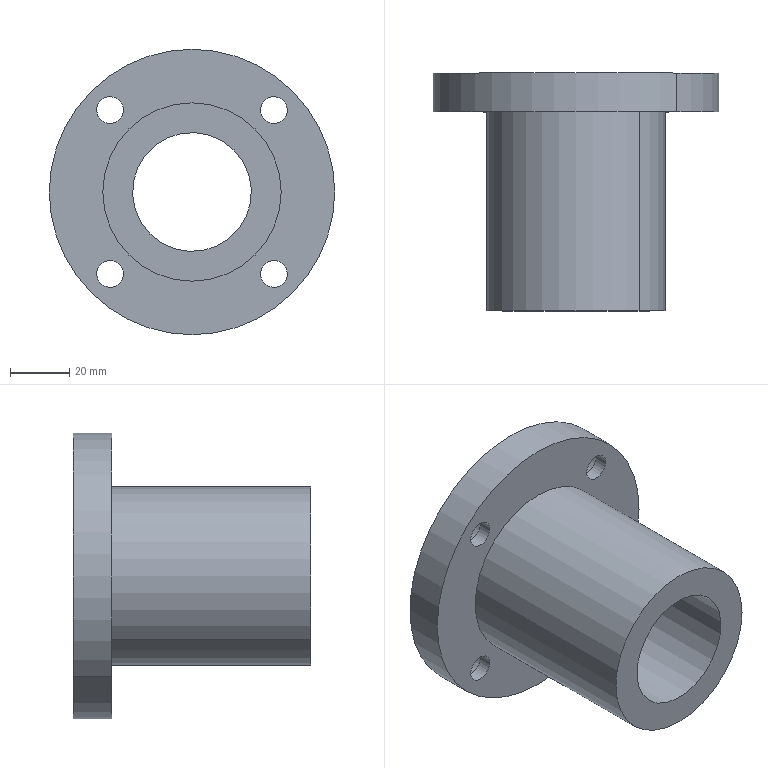Component | SolidWorks | UpperGuidePostAssembly-1_C-LHFR40LinearBearing-1 | 1 solid | 29 faces | box 96 x 80 x 96 mm | volume 175805 mm3 | cylinder 22 | plane 7 | commonest cylinder face diameters 15 x8 9 x8 60 x2 96 x2 40 x2
build123d program:
from build123d import *

# Parameters (mm, degrees)
M8_HEX_SOCKET_HEAD_CAP_SCREW_CBORE1_D           = 9
M8_HEX_SOCKET_HEAD_CAP_SCREW_CBORE1_CBORE_D     = 15
M8_HEX_SOCKET_HEAD_CAP_SCREW_CBORE1_CBORE_DEPTH = 8.6


with BuildPart() as part:
    # Sketch1 → Revolve1 (revolve)
    with BuildSketch(Plane.XY, mode=Mode.PRIVATE) as revolve1_sk:
        Polygon((20, 50.38), (48, 50.38), (48, 37.38), (30, 37.38), (30, -29.62), (20, -29.62), align=None)
    revolve(revolve1_sk.sketch.rotate(Axis((0, -40.515, 0), (0, 1, 0)), 90), axis=Axis((0, -40.515, 0), (0, 1, 0)))

    # M8 Hex Socket Head Cap Screw CBORE1 (through all)
    with Locations(Plane(origin=(0, 50.38, 0), x_dir=(1, 0, 0), z_dir=(0, 1, 0))):
        with Locations((-39, 0), (39, 0), (0, -39), (0, 39)):
            CounterBoreHole(M8_HEX_SOCKET_HEAD_CAP_SCREW_CBORE1_D / 2, M8_HEX_SOCKET_HEAD_CAP_SCREW_CBORE1_CBORE_D / 2, M8_HEX_SOCKET_HEAD_CAP_SCREW_CBORE1_CBORE_DEPTH)


solid = part.part

# Placed as in the assembly
solid = solid.moved(Location((-407.951, 585.89, -225), (180, 45, 180)))
STEP:
#1=COLOUR_RGB('',0.7922,0.8196,0.9333);
#2=FILL_AREA_STYLE_COLOUR('',#1);
#3=FILL_AREA_STYLE('',(#2));
#4=SURFACE_STYLE_FILL_AREA(#3);
#5=SURFACE_SIDE_STYLE('',(#4));
#6=SURFACE_STYLE_USAGE(.BOTH.,#5);
#7=PRESENTATION_STYLE_ASSIGNMENT((#6));
#8=CARTESIAN_POINT('',(-14.767,24.711,-9.735));
#9=VERTEX_POINT('',#8);
#10=CARTESIAN_POINT('',(-15.184,24.711,-10.153));
#11=VERTEX_POINT('',#10);
#12=CARTESIAN_POINT('',(-14.975,24.711,-9.944));
#13=DIRECTION('',(0.,1.,0.));
#14=DIRECTION('',(-0.7071,0.,-0.7071));
#15=AXIS2_PLACEMENT_3D('',#12,#13,#14);
#16=CIRCLE('',#15,0.2953);
#17=EDGE_CURVE('',#9,#11,#16,.T.);
#18=ORIENTED_EDGE('',*,*,#17,.F.);
#19=CARTESIAN_POINT('',(-14.767,25.05,-9.735));
#20=VERTEX_POINT('',#19);
#21=CARTESIAN_POINT('',(-14.767,25.05,-9.735));
#22=DIRECTION('',(0.,1.,0.));
#23=VECTOR('',#22,39.37);
#24=LINE('',#21,#23);
#25=EDGE_CURVE('',#9,#20,#24,.T.);
#26=ORIENTED_EDGE('',*,*,#25,.T.);
#27=CARTESIAN_POINT('',(-15.184,25.05,-10.153));
#28=VERTEX_POINT('',#27);
#29=CARTESIAN_POINT('',(-14.975,25.05,-9.944));
#30=DIRECTION('',(0.,1.,0.));
#31=DIRECTION('',(-0.7071,0.,-0.7071));
#32=AXIS2_PLACEMENT_3D('',#29,#30,#31);
#33=CIRCLE('',#32,0.2953);
#34=EDGE_CURVE('',#20,#28,#33,.T.);
#35=ORIENTED_EDGE('',*,*,#34,.T.);
#36=CARTESIAN_POINT('',(-15.184,25.05,-10.153));
#37=DIRECTION('',(0.,1.,0.));
#38=VECTOR('',#37,39.37);
#39=LINE('',#36,#38);
#40=EDGE_CURVE('',#11,#28,#39,.T.);
#41=ORIENTED_EDGE('',*,*,#40,.F.);
#42=EDGE_LOOP('',(#18,#26,#35,#41));
#43=FACE_OUTER_BOUND('',#42,.T.);
#44=CARTESIAN_POINT('',(-14.975,25.05,-9.944));
#45=DIRECTION('',(0.,1.,0.));
#46=DIRECTION('',(-0.7071,0.,-0.7071));
#47=AXIS2_PLACEMENT_3D('',#44,#45,#46);
#48=CYLINDRICAL_SURFACE('',#47,0.2953);
#49=ADVANCED_FACE('',(#43),#48,.F.);
#50=CARTESIAN_POINT('',(-15.101,24.538,-10.069));
#51=VERTEX_POINT('',#50);
#52=CARTESIAN_POINT('',(-14.85,24.538,-9.819));
#53=VERTEX_POINT('',#52);
#54=CARTESIAN_POINT('',(-14.975,24.538,-9.944));
#55=DIRECTION('',(-0.,-1.,-0.));
#56=DIRECTION('',(0.7071,0.,0.7071));
#57=AXIS2_PLACEMENT_3D('',#54,#55,#56);
#58=CIRCLE('',#57,0.1772);
#59=EDGE_CURVE('',#51,#53,#58,.T.);
#60=ORIENTED_EDGE('',*,*,#59,.T.);
#61=CARTESIAN_POINT('',(-14.85,24.711,-9.819));
#62=VERTEX_POINT('',#61);
#63=CARTESIAN_POINT('',(-14.85,25.05,-9.819));
#64=DIRECTION('',(0.,1.,0.));
#65=VECTOR('',#64,39.37);
#66=LINE('',#63,#65);
#67=EDGE_CURVE('',#53,#62,#66,.T.);
#68=ORIENTED_EDGE('',*,*,#67,.T.);
#69=CARTESIAN_POINT('',(-15.101,24.711,-10.069));
#70=VERTEX_POINT('',#69);
#71=CARTESIAN_POINT('',(-14.975,24.711,-9.944));
#72=DIRECTION('',(0.,1.,0.));
#73=DIRECTION('',(-0.7071,0.,-0.7071));
#74=AXIS2_PLACEMENT_3D('',#71,#72,#73);
#75=CIRCLE('',#74,0.1772);
#76=EDGE_CURVE('',#62,#70,#75,.T.);
#77=ORIENTED_EDGE('',*,*,#76,.T.);
#78=CARTESIAN_POINT('',(-15.101,25.05,-10.069));
#79=DIRECTION('',(0.,1.,0.));
#80=VECTOR('',#79,39.37);
#81=LINE('',#78,#80);
#82=EDGE_CURVE('',#51,#70,#81,.T.);
#83=ORIENTED_EDGE('',*,*,#82,.F.);
#84=EDGE_LOOP('',(#60,#68,#77,#83));
#85=FACE_OUTER_BOUND('',#84,.T.);
#86=CARTESIAN_POINT('',(-14.975,25.05,-9.944));
#87=DIRECTION('',(0.,1.,0.));
#88=DIRECTION('',(-0.7071,0.,-0.7071));
#89=AXIS2_PLACEMENT_3D('',#86,#87,#88);
#90=CYLINDRICAL_SURFACE('',#89,0.1772);
#91=ADVANCED_FACE('',(#85),#90,.F.);
#92=CARTESIAN_POINT('',(-16.938,24.711,-7.564));
#93=VERTEX_POINT('',#92);
#94=CARTESIAN_POINT('',(-17.356,24.711,-7.981));
#95=VERTEX_POINT('',#94);
#96=CARTESIAN_POINT('',(-17.147,24.711,-7.773));
#97=DIRECTION('',(0.,1.,0.));
#98=DIRECTION('',(-0.7071,0.,-0.7071));
#99=AXIS2_PLACEMENT_3D('',#96,#97,#98);
#100=CIRCLE('',#99,0.2953);
#101=EDGE_CURVE('',#93,#95,#100,.T.);
#102=ORIENTED_EDGE('',*,*,#101,.F.);
#103=CARTESIAN_POINT('',(-16.938,25.05,-7.564));
#104=VERTEX_POINT('',#103);
#105=CARTESIAN_POINT('',(-16.938,25.05,-7.564));
#106=DIRECTION('',(0.,1.,0.));
#107=VECTOR('',#106,39.37);
#108=LINE('',#105,#107);
#109=EDGE_CURVE('',#93,#104,#108,.T.);
#110=ORIENTED_EDGE('',*,*,#109,.T.);
#111=CARTESIAN_POINT('',(-17.356,25.05,-7.981));
#112=VERTEX_POINT('',#111);
#113=CARTESIAN_POINT('',(-17.147,25.05,-7.773));
#114=DIRECTION('',(0.,1.,0.));
#115=DIRECTION('',(-0.7071,0.,-0.7071));
#116=AXIS2_PLACEMENT_3D('',#113,#114,#115);
#117=CIRCLE('',#116,0.2953);
#118=EDGE_CURVE('',#104,#112,#117,.T.);
#119=ORIENTED_EDGE('',*,*,#118,.T.);
#120=CARTESIAN_POINT('',(-17.356,25.05,-7.981));
#121=DIRECTION('',(0.,1.,0.));
#122=VECTOR('',#121,39.37);
#123=LINE('',#120,#122);
#124=EDGE_CURVE('',#95,#112,#123,.T.);
#125=ORIENTED_EDGE('',*,*,#124,.F.);
#126=EDGE_LOOP('',(#102,#110,#119,#125));
#127=FACE_OUTER_BOUND('',#126,.T.);
#128=CARTESIAN_POINT('',(-17.147,25.05,-7.773));
#129=DIRECTION('',(0.,1.,0.));
#130=DIRECTION('',(-0.7071,0.,-0.7071));
#131=AXIS2_PLACEMENT_3D('',#128,#129,#130);
#132=CYLINDRICAL_SURFACE('',#131,0.2953);
#133=ADVANCED_FACE('',(#127),#132,.F.);
#134=CARTESIAN_POINT('',(-17.272,24.538,-7.898));
#135=VERTEX_POINT('',#134);
#136=CARTESIAN_POINT('',(-17.021,24.538,-7.647));
#137=VERTEX_POINT('',#136);
#138=CARTESIAN_POINT('',(-17.147,24.538,-7.773));
#139=DIRECTION('',(-0.,-1.,-0.));
#140=DIRECTION('',(0.7071,0.,0.7071));
#141=AXIS2_PLACEMENT_3D('',#138,#139,#140);
#142=CIRCLE('',#141,0.1772);
#143=EDGE_CURVE('',#135,#137,#142,.T.);
#144=ORIENTED_EDGE('',*,*,#143,.T.);
#145=CARTESIAN_POINT('',(-17.021,24.711,-7.647));
#146=VERTEX_POINT('',#145);
#147=CARTESIAN_POINT('',(-17.021,25.05,-7.647));
#148=DIRECTION('',(0.,1.,0.));
#149=VECTOR('',#148,39.37);
#150=LINE('',#147,#149);
#151=EDGE_CURVE('',#137,#146,#150,.T.);
#152=ORIENTED_EDGE('',*,*,#151,.T.);
#153=CARTESIAN_POINT('',(-17.272,24.711,-7.898));
#154=VERTEX_POINT('',#153);
#155=CARTESIAN_POINT('',(-17.147,24.711,-7.773));
#156=DIRECTION('',(0.,1.,0.));
#157=DIRECTION('',(-0.7071,0.,-0.7071));
#158=AXIS2_PLACEMENT_3D('',#155,#156,#157);
#159=CIRCLE('',#158,0.1772);
#160=EDGE_CURVE('',#146,#154,#159,.T.);
#161=ORIENTED_EDGE('',*,*,#160,.T.);
#162=CARTESIAN_POINT('',(-17.272,25.05,-7.898));
#163=DIRECTION('',(0.,1.,0.));
#164=VECTOR('',#163,39.37);
#165=LINE('',#162,#164);
#166=EDGE_CURVE('',#135,#154,#165,.T.);
#167=ORIENTED_EDGE('',*,*,#166,.F.);
#168=EDGE_LOOP('',(#144,#152,#161,#167));
#169=FACE_OUTER_BOUND('',#168,.T.);
#170=CARTESIAN_POINT('',(-17.147,25.05,-7.773));
#171=DIRECTION('',(0.,1.,0.));
#172=DIRECTION('',(-0.7071,0.,-0.7071));
#173=AXIS2_PLACEMENT_3D('',#170,#171,#172);
#174=CYLINDRICAL_SURFACE('',#173,0.1772);
#175=ADVANCED_FACE('',(#169),#174,.F.);
#176=CARTESIAN_POINT('',(-16.938,24.711,-9.735));
#177=VERTEX_POINT('',#176);
#178=CARTESIAN_POINT('',(-17.356,24.711,-10.153));
#179=VERTEX_POINT('',#178);
#180=CARTESIAN_POINT('',(-17.147,24.711,-9.944));
#181=DIRECTION('',(0.,1.,0.));
#182=DIRECTION('',(-0.7071,0.,-0.7071));
#183=AXIS2_PLACEMENT_3D('',#180,#181,#182);
#184=CIRCLE('',#183,0.2953);
#185=EDGE_CURVE('',#177,#179,#184,.T.);
#186=ORIENTED_EDGE('',*,*,#185,.F.);
#187=CARTESIAN_POINT('',(-16.938,25.05,-9.735));
#188=VERTEX_POINT('',#187);
#189=CARTESIAN_POINT('',(-16.938,25.05,-9.735));
#190=DIRECTION('',(0.,1.,0.));
#191=VECTOR('',#190,39.37);
#192=LINE('',#189,#191);
#193=EDGE_CURVE('',#177,#188,#192,.T.);
#194=ORIENTED_EDGE('',*,*,#193,.T.);
#195=CARTESIAN_POINT('',(-17.356,25.05,-10.153));
#196=VERTEX_POINT('',#195);
#197=CARTESIAN_POINT('',(-17.147,25.05,-9.944));
#198=DIRECTION('',(0.,1.,0.));
#199=DIRECTION('',(-0.7071,0.,-0.7071));
#200=AXIS2_PLACEMENT_3D('',#197,#198,#199);
#201=CIRCLE('',#200,0.2953);
#202=EDGE_CURVE('',#188,#196,#201,.T.);
#203=ORIENTED_EDGE('',*,*,#202,.T.);
#204=CARTESIAN_POINT('',(-17.356,25.05,-10.153));
#205=DIRECTION('',(0.,1.,0.));
#206=VECTOR('',#205,39.37);
#207=LINE('',#204,#206);
#208=EDGE_CURVE('',#179,#196,#207,.T.);
#209=ORIENTED_EDGE('',*,*,#208,.F.);
#210=EDGE_LOOP('',(#186,#194,#203,#209));
#211=FACE_OUTER_BOUND('',#210,.T.);
#212=CARTESIAN_POINT('',(-17.147,25.05,-9.944));
#213=DIRECTION('',(0.,1.,0.));
#214=DIRECTION('',(-0.7071,0.,-0.7071));
#215=AXIS2_PLACEMENT_3D('',#212,#213,#214);
#216=CYLINDRICAL_SURFACE('',#215,0.2953);
#217=ADVANCED_FACE('',(#211),#216,.F.);
#218=CARTESIAN_POINT('',(-17.272,24.538,-10.069));
#219=VERTEX_POINT('',#218);
#220=CARTESIAN_POINT('',(-17.021,24.538,-9.819));
#221=VERTEX_POINT('',#220);
#222=CARTESIAN_POINT('',(-17.147,24.538,-9.944));
#223=DIRECTION('',(-0.,-1.,-0.));
#224=DIRECTION('',(0.7071,0.,0.7071));
#225=AXIS2_PLACEMENT_3D('',#222,#223,#224);
#226=CIRCLE('',#225,0.1772);
#227=EDGE_CURVE('',#219,#221,#226,.T.);
#228=ORIENTED_EDGE('',*,*,#227,.T.);
#229=CARTESIAN_POINT('',(-17.021,24.711,-9.819));
#230=VERTEX_POINT('',#229);
#231=CARTESIAN_POINT('',(-17.021,25.05,-9.819));
#232=DIRECTION('',(0.,1.,0.));
#233=VECTOR('',#232,39.37);
#234=LINE('',#231,#233);
#235=EDGE_CURVE('',#221,#230,#234,.T.);
#236=ORIENTED_EDGE('',*,*,#235,.T.);
#237=CARTESIAN_POINT('',(-17.272,24.711,-10.069));
#238=VERTEX_POINT('',#237);
#239=CARTESIAN_POINT('',(-17.147,24.711,-9.944));
#240=DIRECTION('',(0.,1.,0.));
#241=DIRECTION('',(-0.7071,0.,-0.7071));
#242=AXIS2_PLACEMENT_3D('',#239,#240,#241);
#243=CIRCLE('',#242,0.1772);
#244=EDGE_CURVE('',#230,#238,#243,.T.);
#245=ORIENTED_EDGE('',*,*,#244,.T.);
#246=CARTESIAN_POINT('',(-17.272,25.05,-10.069));
#247=DIRECTION('',(0.,1.,0.));
#248=VECTOR('',#247,39.37);
#249=LINE('',#246,#248);
#250=EDGE_CURVE('',#219,#238,#249,.T.);
#251=ORIENTED_EDGE('',*,*,#250,.F.);
#252=EDGE_LOOP('',(#228,#236,#245,#251));
#253=FACE_OUTER_BOUND('',#252,.T.);
#254=CARTESIAN_POINT('',(-17.147,25.05,-9.944));
#255=DIRECTION('',(0.,1.,0.));
#256=DIRECTION('',(-0.7071,0.,-0.7071));
#257=AXIS2_PLACEMENT_3D('',#254,#255,#256);
#258=CYLINDRICAL_SURFACE('',#257,0.1772);
#259=ADVANCED_FACE('',(#253),#258,.F.);
#260=CARTESIAN_POINT('',(-14.767,24.711,-7.564));
#261=VERTEX_POINT('',#260);
#262=CARTESIAN_POINT('',(-15.184,24.711,-7.981));
#263=VERTEX_POINT('',#262);
#264=CARTESIAN_POINT('',(-14.975,24.711,-7.773));
#265=DIRECTION('',(0.,1.,0.));
#266=DIRECTION('',(-0.7071,0.,-0.7071));
#267=AXIS2_PLACEMENT_3D('',#264,#265,#266);
#268=CIRCLE('',#267,0.2953);
#269=EDGE_CURVE('',#261,#263,#268,.T.);
#270=ORIENTED_EDGE('',*,*,#269,.F.);
#271=CARTESIAN_POINT('',(-14.767,25.05,-7.564));
#272=VERTEX_POINT('',#271);
#273=CARTESIAN_POINT('',(-14.767,25.05,-7.564));
#274=DIRECTION('',(0.,1.,0.));
#275=VECTOR('',#274,39.37);
#276=LINE('',#273,#275);
#277=EDGE_CURVE('',#261,#272,#276,.T.);
#278=ORIENTED_EDGE('',*,*,#277,.T.);
#279=CARTESIAN_POINT('',(-15.184,25.05,-7.981));
#280=VERTEX_POINT('',#279);
#281=CARTESIAN_POINT('',(-14.975,25.05,-7.773));
#282=DIRECTION('',(0.,1.,0.));
#283=DIRECTION('',(-0.7071,0.,-0.7071));
#284=AXIS2_PLACEMENT_3D('',#281,#282,#283);
#285=CIRCLE('',#284,0.2953);
#286=EDGE_CURVE('',#272,#280,#285,.T.);
#287=ORIENTED_EDGE('',*,*,#286,.T.);
#288=CARTESIAN_POINT('',(-15.184,25.05,-7.981));
#289=DIRECTION('',(0.,1.,0.));
#290=VECTOR('',#289,39.37);
#291=LINE('',#288,#290);
#292=EDGE_CURVE('',#263,#280,#291,.T.);
#293=ORIENTED_EDGE('',*,*,#292,.F.);
#294=EDGE_LOOP('',(#270,#278,#287,#293));
#295=FACE_OUTER_BOUND('',#294,.T.);
#296=CARTESIAN_POINT('',(-14.975,25.05,-7.773));
#297=DIRECTION('',(0.,1.,0.));
#298=DIRECTION('',(-0.7071,0.,-0.7071));
#299=AXIS2_PLACEMENT_3D('',#296,#297,#298);
#300=CYLINDRICAL_SURFACE('',#299,0.2953);
#301=ADVANCED_FACE('',(#295),#300,.F.);
#302=CARTESIAN_POINT('',(-15.101,24.538,-7.898));
#303=VERTEX_POINT('',#302);
#304=CARTESIAN_POINT('',(-14.85,24.538,-7.647));
#305=VERTEX_POINT('',#304);
#306=CARTESIAN_POINT('',(-14.975,24.538,-7.773));
#307=DIRECTION('',(-0.,-1.,-0.));
#308=DIRECTION('',(0.7071,0.,0.7071));
#309=AXIS2_PLACEMENT_3D('',#306,#307,#308);
#310=CIRCLE('',#309,0.1772);
#311=EDGE_CURVE('',#303,#305,#310,.T.);
#312=ORIENTED_EDGE('',*,*,#311,.T.);
#313=CARTESIAN_POINT('',(-14.85,24.711,-7.647));
#314=VERTEX_POINT('',#313);
#315=CARTESIAN_POINT('',(-14.85,25.05,-7.647));
#316=DIRECTION('',(0.,1.,0.));
#317=VECTOR('',#316,39.37);
#318=LINE('',#315,#317);
#319=EDGE_CURVE('',#305,#314,#318,.T.);
#320=ORIENTED_EDGE('',*,*,#319,.T.);
#321=CARTESIAN_POINT('',(-15.101,24.711,-7.898));
#322=VERTEX_POINT('',#321);
#323=CARTESIAN_POINT('',(-14.975,24.711,-7.773));
#324=DIRECTION('',(0.,1.,0.));
#325=DIRECTION('',(-0.7071,0.,-0.7071));
#326=AXIS2_PLACEMENT_3D('',#323,#324,#325);
#327=CIRCLE('',#326,0.1772);
#328=EDGE_CURVE('',#314,#322,#327,.T.);
#329=ORIENTED_EDGE('',*,*,#328,.T.);
#330=CARTESIAN_POINT('',(-15.101,25.05,-7.898));
#331=DIRECTION('',(0.,1.,0.));
#332=VECTOR('',#331,39.37);
#333=LINE('',#330,#332);
#334=EDGE_CURVE('',#303,#322,#333,.T.);
#335=ORIENTED_EDGE('',*,*,#334,.F.);
#336=EDGE_LOOP('',(#312,#320,#329,#335));
#337=FACE_OUTER_BOUND('',#336,.T.);
#338=CARTESIAN_POINT('',(-14.975,25.05,-7.773));
#339=DIRECTION('',(0.,1.,0.));
#340=DIRECTION('',(-0.7071,0.,-0.7071));
#341=AXIS2_PLACEMENT_3D('',#338,#339,#340);
#342=CYLINDRICAL_SURFACE('',#341,0.1772);
#343=ADVANCED_FACE('',(#337),#342,.F.);
#344=CARTESIAN_POINT('',(-15.226,24.538,-8.023));
#345=VERTEX_POINT('',#344);
#346=CARTESIAN_POINT('',(-16.896,24.538,-9.693));
#347=VERTEX_POINT('',#346);
#348=CARTESIAN_POINT('',(-16.061,24.538,-8.858));
#349=DIRECTION('',(-0.,-1.,-0.));
#350=DIRECTION('',(0.7071,0.,0.7071));
#351=AXIS2_PLACEMENT_3D('',#348,#349,#350);
#352=CIRCLE('',#351,1.181);
#353=EDGE_CURVE('',#345,#347,#352,.T.);
#354=ORIENTED_EDGE('',*,*,#353,.T.);
#355=CARTESIAN_POINT('',(-16.896,21.9,-9.693));
#356=VERTEX_POINT('',#355);
#357=CARTESIAN_POINT('',(-16.896,21.471,-9.693));
#358=DIRECTION('',(-0.,-1.,-0.));
#359=VECTOR('',#358,39.37);
#360=LINE('',#357,#359);
#361=EDGE_CURVE('',#347,#356,#360,.T.);
#362=ORIENTED_EDGE('',*,*,#361,.T.);
#363=CARTESIAN_POINT('',(-15.226,21.9,-8.023));
#364=VERTEX_POINT('',#363);
#365=CARTESIAN_POINT('',(-16.061,21.9,-8.858));
#366=DIRECTION('',(-0.,-1.,-0.));
#367=DIRECTION('',(0.7071,0.,0.7071));
#368=AXIS2_PLACEMENT_3D('',#365,#366,#367);
#369=CIRCLE('',#368,1.181);
#370=EDGE_CURVE('',#364,#356,#369,.T.);
#371=ORIENTED_EDGE('',*,*,#370,.F.);
#372=CARTESIAN_POINT('',(-15.226,21.471,-8.023));
#373=DIRECTION('',(-0.,-1.,-0.));
#374=VECTOR('',#373,39.37);
#375=LINE('',#372,#374);
#376=EDGE_CURVE('',#345,#364,#375,.T.);
#377=ORIENTED_EDGE('',*,*,#376,.F.);
#378=EDGE_LOOP('',(#354,#362,#371,#377));
#379=FACE_OUTER_BOUND('',#378,.T.);
#380=CARTESIAN_POINT('',(-16.061,21.471,-8.858));
#381=DIRECTION('',(-0.,-1.,-0.));
#382=DIRECTION('',(0.7071,0.,0.7071));
#383=AXIS2_PLACEMENT_3D('',#380,#381,#382);
#384=CYLINDRICAL_SURFACE('',#383,1.181);
#385=ADVANCED_FACE('',(#379),#384,.T.);
#386=CARTESIAN_POINT('',(-14.725,25.05,-7.522));
#387=VERTEX_POINT('',#386);
#388=CARTESIAN_POINT('',(-17.397,25.05,-10.195));
#389=VERTEX_POINT('',#388);
#390=CARTESIAN_POINT('',(-16.061,25.05,-8.858));
#391=DIRECTION('',(-0.,-1.,-0.));
#392=DIRECTION('',(0.7071,-0.,0.7071));
#393=AXIS2_PLACEMENT_3D('',#390,#391,#392);
#394=CIRCLE('',#393,1.89);
#395=EDGE_CURVE('',#387,#389,#394,.T.);
#396=ORIENTED_EDGE('',*,*,#395,.T.);
#397=CARTESIAN_POINT('',(-17.397,24.538,-10.195));
#398=VERTEX_POINT('',#397);
#399=CARTESIAN_POINT('',(-17.397,21.471,-10.195));
#400=DIRECTION('',(-0.,-1.,-0.));
#401=VECTOR('',#400,39.37);
#402=LINE('',#399,#401);
#403=EDGE_CURVE('',#389,#398,#402,.T.);
#404=ORIENTED_EDGE('',*,*,#403,.T.);
#405=CARTESIAN_POINT('',(-14.725,24.538,-7.522));
#406=VERTEX_POINT('',#405);
#407=CARTESIAN_POINT('',(-16.061,24.538,-8.858));
#408=DIRECTION('',(-0.,-1.,-0.));
#409=DIRECTION('',(0.7071,-0.,0.7071));
#410=AXIS2_PLACEMENT_3D('',#407,#408,#409);
#411=CIRCLE('',#410,1.89);
#412=EDGE_CURVE('',#406,#398,#411,.T.);
#413=ORIENTED_EDGE('',*,*,#412,.F.);
#414=CARTESIAN_POINT('',(-14.725,21.471,-7.522));
#415=DIRECTION('',(-0.,-1.,-0.));
#416=VECTOR('',#415,39.37);
#417=LINE('',#414,#416);
#418=EDGE_CURVE('',#387,#406,#417,.T.);
#419=ORIENTED_EDGE('',*,*,#418,.F.);
#420=EDGE_LOOP('',(#396,#404,#413,#419));
#421=FACE_OUTER_BOUND('',#420,.T.);
#422=CARTESIAN_POINT('',(-16.061,21.471,-8.858));
#423=DIRECTION('',(-0.,-1.,-0.));
#424=DIRECTION('',(0.7071,-0.,0.7071));
#425=AXIS2_PLACEMENT_3D('',#422,#423,#424);
#426=CYLINDRICAL_SURFACE('',#425,1.89);
#427=ADVANCED_FACE('',(#421),#426,.T.);
#428=CARTESIAN_POINT('',(-16.618,25.05,-9.415));
#429=VERTEX_POINT('',#428);
#430=CARTESIAN_POINT('',(-15.504,25.05,-8.301));
#431=VERTEX_POINT('',#430);
#432=CARTESIAN_POINT('',(-16.061,25.05,-8.858));
#433=DIRECTION('',(-0.,-1.,-0.));
#434=DIRECTION('',(0.7071,0.,0.7071));
#435=AXIS2_PLACEMENT_3D('',#432,#433,#434);
#436=CIRCLE('',#435,0.7874);
#437=EDGE_CURVE('',#429,#431,#436,.T.);
#438=ORIENTED_EDGE('',*,*,#437,.F.);
#439=CARTESIAN_POINT('',(-16.618,21.9,-9.415));
#440=VERTEX_POINT('',#439);
#441=CARTESIAN_POINT('',(-16.618,21.471,-9.415));
#442=DIRECTION('',(-0.,-1.,-0.));
#443=VECTOR('',#442,39.37);
#444=LINE('',#441,#443);
#445=EDGE_CURVE('',#429,#440,#444,.T.);
#446=ORIENTED_EDGE('',*,*,#445,.T.);
#447=CARTESIAN_POINT('',(-15.504,21.9,-8.301));
#448=VERTEX_POINT('',#447);
#449=CARTESIAN_POINT('',(-16.061,21.9,-8.858));
#450=DIRECTION('',(-0.,-1.,-0.));
#451=DIRECTION('',(0.7071,0.,0.7071));
#452=AXIS2_PLACEMENT_3D('',#449,#450,#451);
#453=CIRCLE('',#452,0.7874);
#454=EDGE_CURVE('',#440,#448,#453,.T.);
#455=ORIENTED_EDGE('',*,*,#454,.T.);
#456=CARTESIAN_POINT('',(-15.504,21.471,-8.301));
#457=DIRECTION('',(-0.,-1.,-0.));
#458=VECTOR('',#457,39.37);
#459=LINE('',#456,#458);
#460=EDGE_CURVE('',#431,#448,#459,.T.);
#461=ORIENTED_EDGE('',*,*,#460,.F.);
#462=EDGE_LOOP('',(#438,#446,#455,#461));
#463=FACE_OUTER_BOUND('',#462,.T.);
#464=CARTESIAN_POINT('',(-16.061,21.471,-8.858));
#465=DIRECTION('',(-0.,-1.,-0.));
#466=DIRECTION('',(0.7071,0.,0.7071));
#467=AXIS2_PLACEMENT_3D('',#464,#465,#466);
#468=CYLINDRICAL_SURFACE('',#467,0.7874);
#469=ADVANCED_FACE('',(#463),#468,.F.);
#470=ORIENTED_EDGE('',*,*,#445,.F.);
#471=CARTESIAN_POINT('',(-16.061,25.05,-8.858));
#472=DIRECTION('',(-0.,-1.,-0.));
#473=DIRECTION('',(0.7071,0.,0.7071));
#474=AXIS2_PLACEMENT_3D('',#471,#472,#473);
#475=CIRCLE('',#474,0.7874);
#476=EDGE_CURVE('',#431,#429,#475,.T.);
#477=ORIENTED_EDGE('',*,*,#476,.F.);
#478=ORIENTED_EDGE('',*,*,#460,.T.);
#479=CARTESIAN_POINT('',(-16.061,21.9,-8.858));
#480=DIRECTION('',(-0.,-1.,-0.));
#481=DIRECTION('',(0.7071,0.,0.7071));
#482=AXIS2_PLACEMENT_3D('',#479,#480,#481);
#483=CIRCLE('',#482,0.7874);
#484=EDGE_CURVE('',#448,#440,#483,.T.);
#485=ORIENTED_EDGE('',*,*,#484,.T.);
#486=EDGE_LOOP('',(#470,#477,#478,#485));
#487=FACE_OUTER_BOUND('',#486,.T.);
#488=CARTESIAN_POINT('',(-16.061,21.471,-8.858));
#489=DIRECTION('',(-0.,-1.,-0.));
#490=DIRECTION('',(0.7071,0.,0.7071));
#491=AXIS2_PLACEMENT_3D('',#488,#489,#490);
#492=CYLINDRICAL_SURFACE('',#491,0.7874);
#493=ADVANCED_FACE('',(#487),#492,.F.);
#494=CARTESIAN_POINT('',(-14.975,25.05,-9.944));
#495=DIRECTION('',(0.,1.,0.));
#496=DIRECTION('',(-0.7071,0.,-0.7071));
#497=AXIS2_PLACEMENT_3D('',#494,#495,#496);
#498=CIRCLE('',#497,0.2953);
#499=EDGE_CURVE('',#28,#20,#498,.T.);
#500=ORIENTED_EDGE('',*,*,#499,.F.);
#501=ORIENTED_EDGE('',*,*,#34,.F.);
#502=EDGE_LOOP('',(#500,#501));
#503=FACE_BOUND('',#502,.T.);
#504=CARTESIAN_POINT('',(-17.147,25.05,-7.773));
#505=DIRECTION('',(0.,1.,0.));
#506=DIRECTION('',(-0.7071,0.,-0.7071));
#507=AXIS2_PLACEMENT_3D('',#504,#505,#506);
#508=CIRCLE('',#507,0.2953);
#509=EDGE_CURVE('',#112,#104,#508,.T.);
#510=ORIENTED_EDGE('',*,*,#509,.F.);
#511=ORIENTED_EDGE('',*,*,#118,.F.);
#512=EDGE_LOOP('',(#510,#511));
#513=FACE_BOUND('',#512,.T.);
#514=CARTESIAN_POINT('',(-17.147,25.05,-9.944));
#515=DIRECTION('',(0.,1.,0.));
#516=DIRECTION('',(-0.7071,0.,-0.7071));
#517=AXIS2_PLACEMENT_3D('',#514,#515,#516);
#518=CIRCLE('',#517,0.2953);
#519=EDGE_CURVE('',#196,#188,#518,.T.);
#520=ORIENTED_EDGE('',*,*,#519,.F.);
#521=ORIENTED_EDGE('',*,*,#202,.F.);
#522=EDGE_LOOP('',(#520,#521));
#523=FACE_BOUND('',#522,.T.);
#524=CARTESIAN_POINT('',(-14.975,25.05,-7.773));
#525=DIRECTION('',(0.,1.,0.));
#526=DIRECTION('',(-0.7071,0.,-0.7071));
#527=AXIS2_PLACEMENT_3D('',#524,#525,#526);
#528=CIRCLE('',#527,0.2953);
#529=EDGE_CURVE('',#280,#272,#528,.T.);
#530=ORIENTED_EDGE('',*,*,#529,.F.);
#531=ORIENTED_EDGE('',*,*,#286,.F.);
#532=EDGE_LOOP('',(#530,#531));
#533=FACE_BOUND('',#532,.T.);
#534=ORIENTED_EDGE('',*,*,#476,.T.);
#535=ORIENTED_EDGE('',*,*,#437,.T.);
#536=EDGE_LOOP('',(#534,#535));
#537=FACE_BOUND('',#536,.T.);
#538=ORIENTED_EDGE('',*,*,#395,.F.);
#539=CARTESIAN_POINT('',(-16.061,25.05,-8.858));
#540=DIRECTION('',(-0.,-1.,-0.));
#541=DIRECTION('',(0.7071,-0.,0.7071));
#542=AXIS2_PLACEMENT_3D('',#539,#540,#541);
#543=CIRCLE('',#542,1.89);
#544=EDGE_CURVE('',#389,#387,#543,.T.);
#545=ORIENTED_EDGE('',*,*,#544,.F.);
#546=EDGE_LOOP('',(#538,#545));
#547=FACE_OUTER_BOUND('',#546,.T.);
#548=CARTESIAN_POINT('',(-16.618,25.05,-8.301));
#549=DIRECTION('',(0.,1.,0.));
#550=DIRECTION('',(-0.7071,0.,-0.7071));
#551=AXIS2_PLACEMENT_3D('',#548,#549,#550);
#552=PLANE('',#551);
#553=ADVANCED_FACE('',(#503,#513,#523,#533,#537,#547),#552,.T.);
#554=ORIENTED_EDGE('',*,*,#403,.F.);
#555=ORIENTED_EDGE('',*,*,#544,.T.);
#556=ORIENTED_EDGE('',*,*,#418,.T.);
#557=CARTESIAN_POINT('',(-16.061,24.538,-8.858));
#558=DIRECTION('',(-0.,-1.,-0.));
#559=DIRECTION('',(0.7071,-0.,0.7071));
#560=AXIS2_PLACEMENT_3D('',#557,#558,#559);
#561=CIRCLE('',#560,1.89);
#562=EDGE_CURVE('',#398,#406,#561,.T.);
#563=ORIENTED_EDGE('',*,*,#562,.F.);
#564=EDGE_LOOP('',(#554,#555,#556,#563));
#565=FACE_OUTER_BOUND('',#564,.T.);
#566=CARTESIAN_POINT('',(-16.061,21.471,-8.858));
#567=DIRECTION('',(-0.,-1.,-0.));
#568=DIRECTION('',(0.7071,-0.,0.7071));
#569=AXIS2_PLACEMENT_3D('',#566,#567,#568);
#570=CYLINDRICAL_SURFACE('',#569,1.89);
#571=ADVANCED_FACE('',(#565),#570,.T.);
#572=ORIENTED_EDGE('',*,*,#59,.F.);
#573=CARTESIAN_POINT('',(-14.975,24.538,-9.944));
#574=DIRECTION('',(-0.,-1.,-0.));
#575=DIRECTION('',(0.7071,0.,0.7071));
#576=AXIS2_PLACEMENT_3D('',#573,#574,#575);
#577=CIRCLE('',#576,0.1772);
#578=EDGE_CURVE('',#53,#51,#577,.T.);
#579=ORIENTED_EDGE('',*,*,#578,.F.);
#580=EDGE_LOOP('',(#572,#579));
#581=FACE_BOUND('',#580,.T.);
#582=ORIENTED_EDGE('',*,*,#143,.F.);
#583=CARTESIAN_POINT('',(-17.147,24.538,-7.773));
#584=DIRECTION('',(-0.,-1.,-0.));
#585=DIRECTION('',(0.7071,0.,0.7071));
#586=AXIS2_PLACEMENT_3D('',#583,#584,#585);
#587=CIRCLE('',#586,0.1772);
#588=EDGE_CURVE('',#137,#135,#587,.T.);
#589=ORIENTED_EDGE('',*,*,#588,.F.);
#590=EDGE_LOOP('',(#582,#589));
#591=FACE_BOUND('',#590,.T.);
#592=ORIENTED_EDGE('',*,*,#227,.F.);
#593=CARTESIAN_POINT('',(-17.147,24.538,-9.944));
#594=DIRECTION('',(-0.,-1.,-0.));
#595=DIRECTION('',(0.7071,0.,0.7071));
#596=AXIS2_PLACEMENT_3D('',#593,#594,#595);
#597=CIRCLE('',#596,0.1772);
#598=EDGE_CURVE('',#221,#219,#597,.T.);
#599=ORIENTED_EDGE('',*,*,#598,.F.);
#600=EDGE_LOOP('',(#592,#599));
#601=FACE_BOUND('',#600,.T.);
#602=ORIENTED_EDGE('',*,*,#311,.F.);
#603=CARTESIAN_POINT('',(-14.975,24.538,-7.773));
#604=DIRECTION('',(-0.,-1.,-0.));
#605=DIRECTION('',(0.7071,0.,0.7071));
#606=AXIS2_PLACEMENT_3D('',#603,#604,#605);
#607=CIRCLE('',#606,0.1772);
#608=EDGE_CURVE('',#305,#303,#607,.T.);
#609=ORIENTED_EDGE('',*,*,#608,.F.);
#610=EDGE_LOOP('',(#602,#609));
#611=FACE_BOUND('',#610,.T.);
#612=ORIENTED_EDGE('',*,*,#412,.T.);
#613=ORIENTED_EDGE('',*,*,#562,.T.);
#614=EDGE_LOOP('',(#612,#613));
#615=FACE_OUTER_BOUND('',#614,.T.);
#616=ORIENTED_EDGE('',*,*,#353,.F.);
#617=CARTESIAN_POINT('',(-16.061,24.538,-8.858));
#618=DIRECTION('',(-0.,-1.,-0.));
#619=DIRECTION('',(0.7071,0.,0.7071));
#620=AXIS2_PLACEMENT_3D('',#617,#618,#619);
#621=CIRCLE('',#620,1.181);
#622=EDGE_CURVE('',#347,#345,#621,.T.);
#623=ORIENTED_EDGE('',*,*,#622,.F.);
#624=EDGE_LOOP('',(#616,#623));
#625=FACE_BOUND('',#624,.T.);
#626=CARTESIAN_POINT('',(-17.397,24.538,-7.522));
#627=DIRECTION('',(-0.,-1.,-0.));
#628=DIRECTION('',(0.7071,-0.,0.7071));
#629=AXIS2_PLACEMENT_3D('',#626,#627,#628);
#630=PLANE('',#629);
#631=ADVANCED_FACE('',(#581,#591,#601,#611,#615,#625),#630,.T.);
#632=ORIENTED_EDGE('',*,*,#361,.F.);
#633=ORIENTED_EDGE('',*,*,#622,.T.);
#634=ORIENTED_EDGE('',*,*,#376,.T.);
#635=CARTESIAN_POINT('',(-16.061,21.9,-8.858));
#636=DIRECTION('',(-0.,-1.,-0.));
#637=DIRECTION('',(0.7071,0.,0.7071));
#638=AXIS2_PLACEMENT_3D('',#635,#636,#637);
#639=CIRCLE('',#638,1.181);
#640=EDGE_CURVE('',#356,#364,#639,.T.);
#641=ORIENTED_EDGE('',*,*,#640,.F.);
#642=EDGE_LOOP('',(#632,#633,#634,#641));
#643=FACE_OUTER_BOUND('',#642,.T.);
#644=CARTESIAN_POINT('',(-16.061,21.471,-8.858));
#645=DIRECTION('',(-0.,-1.,-0.));
#646=DIRECTION('',(0.7071,0.,0.7071));
#647=AXIS2_PLACEMENT_3D('',#644,#645,#646);
#648=CYLINDRICAL_SURFACE('',#647,1.181);
#649=ADVANCED_FACE('',(#643),#648,.T.);
#650=ORIENTED_EDGE('',*,*,#370,.T.);
#651=ORIENTED_EDGE('',*,*,#640,.T.);
#652=EDGE_LOOP('',(#650,#651));
#653=FACE_OUTER_BOUND('',#652,.T.);
#654=ORIENTED_EDGE('',*,*,#484,.F.);
#655=ORIENTED_EDGE('',*,*,#454,.F.);
#656=EDGE_LOOP('',(#654,#655));
#657=FACE_BOUND('',#656,.T.);
#658=CARTESIAN_POINT('',(-16.896,21.9,-8.023));
#659=DIRECTION('',(-0.,-1.,-0.));
#660=DIRECTION('',(0.7071,-0.,0.7071));
#661=AXIS2_PLACEMENT_3D('',#658,#659,#660);
#662=PLANE('',#661);
#663=ADVANCED_FACE('',(#653,#657),#662,.T.);
#664=ORIENTED_EDGE('',*,*,#319,.F.);
#665=ORIENTED_EDGE('',*,*,#608,.T.);
#666=ORIENTED_EDGE('',*,*,#334,.T.);
#667=CARTESIAN_POINT('',(-14.975,24.711,-7.773));
#668=DIRECTION('',(0.,1.,0.));
#669=DIRECTION('',(-0.7071,0.,-0.7071));
#670=AXIS2_PLACEMENT_3D('',#667,#668,#669);
#671=CIRCLE('',#670,0.1772);
#672=EDGE_CURVE('',#322,#314,#671,.T.);
#673=ORIENTED_EDGE('',*,*,#672,.T.);
#674=EDGE_LOOP('',(#664,#665,#666,#673));
#675=FACE_OUTER_BOUND('',#674,.T.);
#676=CARTESIAN_POINT('',(-14.975,25.05,-7.773));
#677=DIRECTION('',(0.,1.,0.));
#678=DIRECTION('',(-0.7071,0.,-0.7071));
#679=AXIS2_PLACEMENT_3D('',#676,#677,#678);
#680=CYLINDRICAL_SURFACE('',#679,0.1772);
#681=ADVANCED_FACE('',(#675),#680,.F.);
#682=ORIENTED_EDGE('',*,*,#672,.F.);
#683=ORIENTED_EDGE('',*,*,#328,.F.);
#684=EDGE_LOOP('',(#682,#683));
#685=FACE_BOUND('',#684,.T.);
#686=CARTESIAN_POINT('',(-14.975,24.711,-7.773));
#687=DIRECTION('',(0.,1.,0.));
#688=DIRECTION('',(-0.7071,0.,-0.7071));
#689=AXIS2_PLACEMENT_3D('',#686,#687,#688);
#690=CIRCLE('',#689,0.2953);
#691=EDGE_CURVE('',#263,#261,#690,.T.);
#692=ORIENTED_EDGE('',*,*,#691,.T.);
#693=ORIENTED_EDGE('',*,*,#269,.T.);
#694=EDGE_LOOP('',(#692,#693));
#695=FACE_OUTER_BOUND('',#694,.T.);
#696=CARTESIAN_POINT('',(-15.101,24.711,-7.647));
#697=DIRECTION('',(-0.,-1.,-0.));
#698=DIRECTION('',(0.7071,-0.,0.7071));
#699=AXIS2_PLACEMENT_3D('',#696,#697,#698);
#700=PLANE('',#699);
#701=ADVANCED_FACE('',(#685,#695),#700,.F.);
#702=ORIENTED_EDGE('',*,*,#277,.F.);
#703=ORIENTED_EDGE('',*,*,#691,.F.);
#704=ORIENTED_EDGE('',*,*,#292,.T.);
#705=ORIENTED_EDGE('',*,*,#529,.T.);
#706=EDGE_LOOP('',(#702,#703,#704,#705));
#707=FACE_OUTER_BOUND('',#706,.T.);
#708=CARTESIAN_POINT('',(-14.975,25.05,-7.773));
#709=DIRECTION('',(0.,1.,0.));
#710=DIRECTION('',(-0.7071,0.,-0.7071));
#711=AXIS2_PLACEMENT_3D('',#708,#709,#710);
#712=CYLINDRICAL_SURFACE('',#711,0.2953);
#713=ADVANCED_FACE('',(#707),#712,.F.);
#714=ORIENTED_EDGE('',*,*,#235,.F.);
#715=ORIENTED_EDGE('',*,*,#598,.T.);
#716=ORIENTED_EDGE('',*,*,#250,.T.);
#717=CARTESIAN_POINT('',(-17.147,24.711,-9.944));
#718=DIRECTION('',(0.,1.,0.));
#719=DIRECTION('',(-0.7071,0.,-0.7071));
#720=AXIS2_PLACEMENT_3D('',#717,#718,#719);
#721=CIRCLE('',#720,0.1772);
#722=EDGE_CURVE('',#238,#230,#721,.T.);
#723=ORIENTED_EDGE('',*,*,#722,.T.);
#724=EDGE_LOOP('',(#714,#715,#716,#723));
#725=FACE_OUTER_BOUND('',#724,.T.);
#726=CARTESIAN_POINT('',(-17.147,25.05,-9.944));
#727=DIRECTION('',(0.,1.,0.));
#728=DIRECTION('',(-0.7071,0.,-0.7071));
#729=AXIS2_PLACEMENT_3D('',#726,#727,#728);
#730=CYLINDRICAL_SURFACE('',#729,0.1772);
#731=ADVANCED_FACE('',(#725),#730,.F.);
#732=ORIENTED_EDGE('',*,*,#722,.F.);
#733=ORIENTED_EDGE('',*,*,#244,.F.);
#734=EDGE_LOOP('',(#732,#733));
#735=FACE_BOUND('',#734,.T.);
#736=CARTESIAN_POINT('',(-17.147,24.711,-9.944));
#737=DIRECTION('',(0.,1.,0.));
#738=DIRECTION('',(-0.7071,0.,-0.7071));
#739=AXIS2_PLACEMENT_3D('',#736,#737,#738);
#740=CIRCLE('',#739,0.2953);
#741=EDGE_CURVE('',#179,#177,#740,.T.);
#742=ORIENTED_EDGE('',*,*,#741,.T.);
#743=ORIENTED_EDGE('',*,*,#185,.T.);
#744=EDGE_LOOP('',(#742,#743));
#745=FACE_OUTER_BOUND('',#744,.T.);
#746=CARTESIAN_POINT('',(-17.272,24.711,-9.819));
#747=DIRECTION('',(-0.,-1.,-0.));
#748=DIRECTION('',(0.7071,-0.,0.7071));
#749=AXIS2_PLACEMENT_3D('',#746,#747,#748);
#750=PLANE('',#749);
#751=ADVANCED_FACE('',(#735,#745),#750,.F.);
#752=ORIENTED_EDGE('',*,*,#193,.F.);
#753=ORIENTED_EDGE('',*,*,#741,.F.);
#754=ORIENTED_EDGE('',*,*,#208,.T.);
#755=ORIENTED_EDGE('',*,*,#519,.T.);
#756=EDGE_LOOP('',(#752,#753,#754,#755));
#757=FACE_OUTER_BOUND('',#756,.T.);
#758=CARTESIAN_POINT('',(-17.147,25.05,-9.944));
#759=DIRECTION('',(0.,1.,0.));
#760=DIRECTION('',(-0.7071,0.,-0.7071));
#761=AXIS2_PLACEMENT_3D('',#758,#759,#760);
#762=CYLINDRICAL_SURFACE('',#761,0.2953);
#763=ADVANCED_FACE('',(#757),#762,.F.);
#764=ORIENTED_EDGE('',*,*,#151,.F.);
#765=ORIENTED_EDGE('',*,*,#588,.T.);
#766=ORIENTED_EDGE('',*,*,#166,.T.);
#767=CARTESIAN_POINT('',(-17.147,24.711,-7.773));
#768=DIRECTION('',(0.,1.,0.));
#769=DIRECTION('',(-0.7071,0.,-0.7071));
#770=AXIS2_PLACEMENT_3D('',#767,#768,#769);
#771=CIRCLE('',#770,0.1772);
#772=EDGE_CURVE('',#154,#146,#771,.T.);
#773=ORIENTED_EDGE('',*,*,#772,.T.);
#774=EDGE_LOOP('',(#764,#765,#766,#773));
#775=FACE_OUTER_BOUND('',#774,.T.);
#776=CARTESIAN_POINT('',(-17.147,25.05,-7.773));
#777=DIRECTION('',(0.,1.,0.));
#778=DIRECTION('',(-0.7071,0.,-0.7071));
#779=AXIS2_PLACEMENT_3D('',#776,#777,#778);
#780=CYLINDRICAL_SURFACE('',#779,0.1772);
#781=ADVANCED_FACE('',(#775),#780,.F.);
#782=ORIENTED_EDGE('',*,*,#772,.F.);
#783=ORIENTED_EDGE('',*,*,#160,.F.);
#784=EDGE_LOOP('',(#782,#783));
#785=FACE_BOUND('',#784,.T.);
#786=CARTESIAN_POINT('',(-17.147,24.711,-7.773));
#787=DIRECTION('',(0.,1.,0.));
#788=DIRECTION('',(-0.7071,0.,-0.7071));
#789=AXIS2_PLACEMENT_3D('',#786,#787,#788);
#790=CIRCLE('',#789,0.2953);
#791=EDGE_CURVE('',#95,#93,#790,.T.);
#792=ORIENTED_EDGE('',*,*,#791,.T.);
#793=ORIENTED_EDGE('',*,*,#101,.T.);
#794=EDGE_LOOP('',(#792,#793));
#795=FACE_OUTER_BOUND('',#794,.T.);
#796=CARTESIAN_POINT('',(-17.272,24.711,-7.647));
#797=DIRECTION('',(-0.,-1.,-0.));
#798=DIRECTION('',(0.7071,-0.,0.7071));
#799=AXIS2_PLACEMENT_3D('',#796,#797,#798);
#800=PLANE('',#799);
#801=ADVANCED_FACE('',(#785,#795),#800,.F.);
#802=ORIENTED_EDGE('',*,*,#109,.F.);
#803=ORIENTED_EDGE('',*,*,#791,.F.);
#804=ORIENTED_EDGE('',*,*,#124,.T.);
#805=ORIENTED_EDGE('',*,*,#509,.T.);
#806=EDGE_LOOP('',(#802,#803,#804,#805));
#807=FACE_OUTER_BOUND('',#806,.T.);
#808=CARTESIAN_POINT('',(-17.147,25.05,-7.773));
#809=DIRECTION('',(0.,1.,0.));
#810=DIRECTION('',(-0.7071,0.,-0.7071));
#811=AXIS2_PLACEMENT_3D('',#808,#809,#810);
#812=CYLINDRICAL_SURFACE('',#811,0.2953);
#813=ADVANCED_FACE('',(#807),#812,.F.);
#814=ORIENTED_EDGE('',*,*,#67,.F.);
#815=ORIENTED_EDGE('',*,*,#578,.T.);
#816=ORIENTED_EDGE('',*,*,#82,.T.);
#817=CARTESIAN_POINT('',(-14.975,24.711,-9.944));
#818=DIRECTION('',(0.,1.,0.));
#819=DIRECTION('',(-0.7071,0.,-0.7071));
#820=AXIS2_PLACEMENT_3D('',#817,#818,#819);
#821=CIRCLE('',#820,0.1772);
#822=EDGE_CURVE('',#70,#62,#821,.T.);
#823=ORIENTED_EDGE('',*,*,#822,.T.);
#824=EDGE_LOOP('',(#814,#815,#816,#823));
#825=FACE_OUTER_BOUND('',#824,.T.);
#826=CARTESIAN_POINT('',(-14.975,25.05,-9.944));
#827=DIRECTION('',(0.,1.,0.));
#828=DIRECTION('',(-0.7071,0.,-0.7071));
#829=AXIS2_PLACEMENT_3D('',#826,#827,#828);
#830=CYLINDRICAL_SURFACE('',#829,0.1772);
#831=ADVANCED_FACE('',(#825),#830,.F.);
#832=ORIENTED_EDGE('',*,*,#822,.F.);
#833=ORIENTED_EDGE('',*,*,#76,.F.);
#834=EDGE_LOOP('',(#832,#833));
#835=FACE_BOUND('',#834,.T.);
#836=CARTESIAN_POINT('',(-14.975,24.711,-9.944));
#837=DIRECTION('',(0.,1.,0.));
#838=DIRECTION('',(-0.7071,0.,-0.7071));
#839=AXIS2_PLACEMENT_3D('',#836,#837,#838);
#840=CIRCLE('',#839,0.2953);
#841=EDGE_CURVE('',#11,#9,#840,.T.);
#842=ORIENTED_EDGE('',*,*,#841,.T.);
#843=ORIENTED_EDGE('',*,*,#17,.T.);
#844=EDGE_LOOP('',(#842,#843));
#845=FACE_OUTER_BOUND('',#844,.T.);
#846=CARTESIAN_POINT('',(-15.101,24.711,-9.819));
#847=DIRECTION('',(-0.,-1.,-0.));
#848=DIRECTION('',(0.7071,-0.,0.7071));
#849=AXIS2_PLACEMENT_3D('',#846,#847,#848);
#850=PLANE('',#849);
#851=ADVANCED_FACE('',(#835,#845),#850,.F.);
#852=ORIENTED_EDGE('',*,*,#25,.F.);
#853=ORIENTED_EDGE('',*,*,#841,.F.);
#854=ORIENTED_EDGE('',*,*,#40,.T.);
#855=ORIENTED_EDGE('',*,*,#499,.T.);
#856=EDGE_LOOP('',(#852,#853,#854,#855));
#857=FACE_OUTER_BOUND('',#856,.T.);
#858=CARTESIAN_POINT('',(-14.975,25.05,-9.944));
#859=DIRECTION('',(0.,1.,0.));
#860=DIRECTION('',(-0.7071,0.,-0.7071));
#861=AXIS2_PLACEMENT_3D('',#858,#859,#860);
#862=CYLINDRICAL_SURFACE('',#861,0.2953);
#863=ADVANCED_FACE('',(#857),#862,.F.);
#864=CLOSED_SHELL('',(#49,#91,#133,#175,#217,#259,#301,#343,#385,#427,#469,#493,#553,#571,#631,#649,#663,#681,#701,#713,#731,#751,#763,#781,#801,#813,#831,#851,#863));
#865=MANIFOLD_SOLID_BREP('',#864);
#866=STYLED_ITEM('',(#7),#865);
#867=PRESENTATION_LAYER_ASSIGNMENT('','',(#866));
#868=CARTESIAN_POINT('',(0.,0.,0.));
#869=DIRECTION('',(0.,0.,1.));
#870=DIRECTION('',(1.,0.,0.));
#871=AXIS2_PLACEMENT_3D('',#868,#869,#870);
#872=(LENGTH_UNIT()NAMED_UNIT(*)SI_UNIT($,.METRE.));
#873=LENGTH_MEASURE_WITH_UNIT(LENGTH_MEASURE(0.0254),#872);
#874=DIMENSIONAL_EXPONENTS(1.,0.,0.,0.,0.,0.,0.);
#875=(CONVERSION_BASED_UNIT('',#873)LENGTH_UNIT()NAMED_UNIT(#874));
#876=UNCERTAINTY_MEASURE_WITH_UNIT(LENGTH_MEASURE(0.00001),#875,'','');
#877=(NAMED_UNIT(*)PLANE_ANGLE_UNIT()SI_UNIT($,.RADIAN.));
#878=(NAMED_UNIT(*)SI_UNIT($,.STERADIAN.)SOLID_ANGLE_UNIT());
#879=(GEOMETRIC_REPRESENTATION_CONTEXT(3)GLOBAL_UNCERTAINTY_ASSIGNED_CONTEXT((#876))GLOBAL_UNIT_ASSIGNED_CONTEXT((#875,#877,#878))REPRESENTATION_CONTEXT('',''));
#880=ADVANCED_BREP_SHAPE_REPRESENTATION('',(#865,#871),#879);
#881=(LENGTH_UNIT()NAMED_UNIT(*)SI_UNIT($,.METRE.));
#882=LENGTH_MEASURE_WITH_UNIT(LENGTH_MEASURE(0.0254),#881);
#883=DIMENSIONAL_EXPONENTS(1.,0.,0.,0.,0.,0.,0.);
#884=(CONVERSION_BASED_UNIT('',#882)LENGTH_UNIT()NAMED_UNIT(#883));
#885=UNCERTAINTY_MEASURE_WITH_UNIT(LENGTH_MEASURE(0.00001),#884,'','');
#886=(NAMED_UNIT(*)PLANE_ANGLE_UNIT()SI_UNIT($,.RADIAN.));
#887=(NAMED_UNIT(*)SI_UNIT($,.STERADIAN.)SOLID_ANGLE_UNIT());
#888=(GEOMETRIC_REPRESENTATION_CONTEXT(3)GLOBAL_UNCERTAINTY_ASSIGNED_CONTEXT((#885))GLOBAL_UNIT_ASSIGNED_CONTEXT((#884,#886,#887))REPRESENTATION_CONTEXT('',''));
#889=MECHANICAL_DESIGN_GEOMETRIC_PRESENTATION_REPRESENTATION('',(#866),#888);